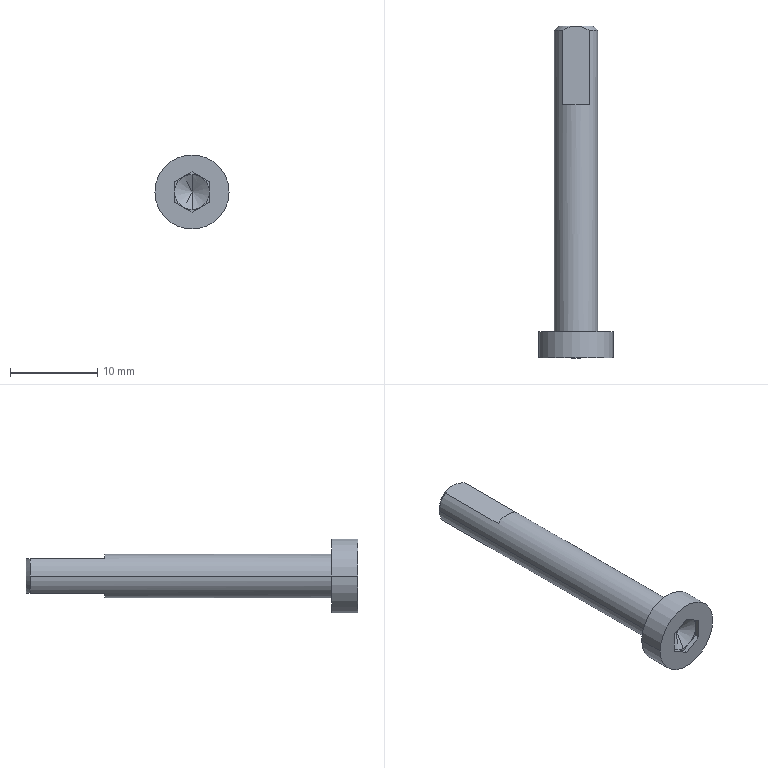Component | SolidWorks | 18M5-L35StainlessSteelScrew-1 | 1 solid | 28 faces | box 8.5 x 38 x 8.5 mm | volume 826 mm3 | plane 19 | cone 5 | cylinder 4 | commonest cylinder face diameters 5 x2 8.5 x2 | material SUS304
STEP:
#1=COLOUR_RGB('',0.7922,0.8196,0.9333);
#2=FILL_AREA_STYLE_COLOUR('',#1);
#3=FILL_AREA_STYLE('',(#2));
#4=SURFACE_STYLE_FILL_AREA(#3);
#5=SURFACE_SIDE_STYLE('',(#4));
#6=SURFACE_STYLE_USAGE(.BOTH.,#5);
#7=PRESENTATION_STYLE_ASSIGNMENT((#6));
#8=CARTESIAN_POINT('',(-0.5354,0.004919,3.11));
#9=VERTEX_POINT('',#8);
#10=CARTESIAN_POINT('',(-0.5354,-0.04054,3.031));
#11=VERTEX_POINT('',#10);
#12=CARTESIAN_POINT('',(-0.5354,-0.04054,3.031));
#13=DIRECTION('',(0.,-0.5,-0.866));
#14=VECTOR('',#13,39.37);
#15=LINE('',#12,#14);
#16=EDGE_CURVE('',#9,#11,#15,.T.);
#17=ORIENTED_EDGE('',*,*,#16,.F.);
#18=CARTESIAN_POINT('',(-0.5354,-0.04054,3.189));
#19=VERTEX_POINT('',#18);
#20=CARTESIAN_POINT('',(-0.5354,-0.04054,3.189));
#21=DIRECTION('',(0.,-0.5,0.866));
#22=VECTOR('',#21,39.37);
#23=LINE('',#20,#22);
#24=EDGE_CURVE('',#9,#19,#23,.T.);
#25=ORIENTED_EDGE('',*,*,#24,.T.);
#26=CARTESIAN_POINT('',(-0.5748,-0.04054,3.178));
#27=VERTEX_POINT('',#26);
#28=CARTESIAN_POINT('',(-0.5354,-0.04054,3.11));
#29=DIRECTION('',(-0.,1.,-0.));
#30=DIRECTION('',(0.,-0.,-1.));
#31=AXIS2_PLACEMENT_3D('',#28,#29,#30);
#32=CIRCLE('',#31,0.07874);
#33=EDGE_CURVE('',#27,#19,#32,.T.);
#34=ORIENTED_EDGE('',*,*,#33,.F.);
#35=CARTESIAN_POINT('',(-0.6142,-0.04054,3.11));
#36=VERTEX_POINT('',#35);
#37=CARTESIAN_POINT('',(-0.5354,-0.04054,3.11));
#38=DIRECTION('',(-0.,1.,-0.));
#39=DIRECTION('',(-0.,-0.,-1.));
#40=AXIS2_PLACEMENT_3D('',#37,#38,#39);
#41=CIRCLE('',#40,0.07874);
#42=EDGE_CURVE('',#36,#27,#41,.T.);
#43=ORIENTED_EDGE('',*,*,#42,.F.);
#44=CARTESIAN_POINT('',(-0.5748,-0.04054,3.042));
#45=VERTEX_POINT('',#44);
#46=CARTESIAN_POINT('',(-0.5354,-0.04054,3.11));
#47=DIRECTION('',(-0.,1.,-0.));
#48=DIRECTION('',(0.,-0.,-1.));
#49=AXIS2_PLACEMENT_3D('',#46,#47,#48);
#50=CIRCLE('',#49,0.07874);
#51=EDGE_CURVE('',#45,#36,#50,.T.);
#52=ORIENTED_EDGE('',*,*,#51,.F.);
#53=CARTESIAN_POINT('',(-0.5354,-0.04054,3.11));
#54=DIRECTION('',(-0.,1.,-0.));
#55=DIRECTION('',(0.,-0.,-1.));
#56=AXIS2_PLACEMENT_3D('',#53,#54,#55);
#57=CIRCLE('',#56,0.07874);
#58=EDGE_CURVE('',#11,#45,#57,.T.);
#59=ORIENTED_EDGE('',*,*,#58,.F.);
#60=EDGE_LOOP('',(#17,#25,#34,#43,#52,#59));
#61=FACE_OUTER_BOUND('',#60,.T.);
#62=CARTESIAN_POINT('',(-0.5354,-0.04054,3.11));
#63=DIRECTION('',(0.,-1.,0.));
#64=DIRECTION('',(0.,-0.,-1.));
#65=AXIS2_PLACEMENT_3D('',#62,#63,#64);
#66=CONICAL_SURFACE('',#65,0.07874,1.047);
#67=ADVANCED_FACE('',(#61),#66,.F.);
#68=CARTESIAN_POINT('',(-0.5945,1.417,3.189));
#69=VERTEX_POINT('',#68);
#70=CARTESIAN_POINT('',(-0.6338,1.417,3.11));
#71=VERTEX_POINT('',#70);
#72=CARTESIAN_POINT('',(-0.5354,1.417,3.11));
#73=DIRECTION('',(0.,-1.,0.));
#74=DIRECTION('',(1.,0.,0.));
#75=AXIS2_PLACEMENT_3D('',#72,#73,#74);
#76=CIRCLE('',#75,0.09843);
#77=EDGE_CURVE('',#69,#71,#76,.T.);
#78=ORIENTED_EDGE('',*,*,#77,.T.);
#79=CARTESIAN_POINT('',(-0.6338,0.05788,3.11));
#80=VERTEX_POINT('',#79);
#81=CARTESIAN_POINT('',(-0.6338,1.436,3.11));
#82=DIRECTION('',(0.,-1.,0.));
#83=VECTOR('',#82,39.37);
#84=LINE('',#81,#83);
#85=EDGE_CURVE('',#71,#80,#84,.T.);
#86=ORIENTED_EDGE('',*,*,#85,.T.);
#87=CARTESIAN_POINT('',(-0.437,0.05788,3.11));
#88=VERTEX_POINT('',#87);
#89=CARTESIAN_POINT('',(-0.5354,0.05788,3.11));
#90=DIRECTION('',(-0.,1.,-0.));
#91=DIRECTION('',(1.,0.,0.));
#92=AXIS2_PLACEMENT_3D('',#89,#90,#91);
#93=CIRCLE('',#92,0.09843);
#94=EDGE_CURVE('',#80,#88,#93,.T.);
#95=ORIENTED_EDGE('',*,*,#94,.T.);
#96=CARTESIAN_POINT('',(-0.437,1.417,3.11));
#97=VERTEX_POINT('',#96);
#98=CARTESIAN_POINT('',(-0.437,1.436,3.11));
#99=DIRECTION('',(0.,-1.,0.));
#100=VECTOR('',#99,39.37);
#101=LINE('',#98,#100);
#102=EDGE_CURVE('',#97,#88,#101,.T.);
#103=ORIENTED_EDGE('',*,*,#102,.F.);
#104=CARTESIAN_POINT('',(-0.4764,1.417,3.189));
#105=VERTEX_POINT('',#104);
#106=CARTESIAN_POINT('',(-0.5354,1.417,3.11));
#107=DIRECTION('',(0.,-1.,0.));
#108=DIRECTION('',(1.,0.,0.));
#109=AXIS2_PLACEMENT_3D('',#106,#107,#108);
#110=CIRCLE('',#109,0.09843);
#111=EDGE_CURVE('',#97,#105,#110,.T.);
#112=ORIENTED_EDGE('',*,*,#111,.T.);
#113=CARTESIAN_POINT('',(-0.4764,1.082,3.189));
#114=VERTEX_POINT('',#113);
#115=CARTESIAN_POINT('',(-0.4764,1.082,3.189));
#116=DIRECTION('',(-0.,1.,-0.));
#117=VECTOR('',#116,39.37);
#118=LINE('',#115,#117);
#119=EDGE_CURVE('',#114,#105,#118,.T.);
#120=ORIENTED_EDGE('',*,*,#119,.F.);
#121=CARTESIAN_POINT('',(-0.5945,1.082,3.189));
#122=VERTEX_POINT('',#121);
#123=CARTESIAN_POINT('',(-0.5354,1.082,3.11));
#124=DIRECTION('',(-0.,1.,-0.));
#125=DIRECTION('',(-1.,0.,0.));
#126=AXIS2_PLACEMENT_3D('',#123,#124,#125);
#127=CIRCLE('',#126,0.09843);
#128=EDGE_CURVE('',#122,#114,#127,.T.);
#129=ORIENTED_EDGE('',*,*,#128,.F.);
#130=CARTESIAN_POINT('',(-0.5945,1.082,3.189));
#131=DIRECTION('',(-0.,1.,-0.));
#132=VECTOR('',#131,39.37);
#133=LINE('',#130,#132);
#134=EDGE_CURVE('',#122,#69,#133,.T.);
#135=ORIENTED_EDGE('',*,*,#134,.T.);
#136=EDGE_LOOP('',(#78,#86,#95,#103,#112,#120,#129,#135));
#137=FACE_OUTER_BOUND('',#136,.T.);
#138=CARTESIAN_POINT('',(-0.5354,1.436,3.11));
#139=DIRECTION('',(0.,-1.,0.));
#140=DIRECTION('',(1.,0.,0.));
#141=AXIS2_PLACEMENT_3D('',#138,#139,#140);
#142=CYLINDRICAL_SURFACE('',#141,0.09843);
#143=ADVANCED_FACE('',(#137),#142,.T.);
#144=CARTESIAN_POINT('',(-0.5277,1.436,3.031));
#145=VERTEX_POINT('',#144);
#146=CARTESIAN_POINT('',(-0.4563,1.436,3.11));
#147=VERTEX_POINT('',#146);
#148=CARTESIAN_POINT('',(-0.5354,1.436,3.11));
#149=DIRECTION('',(0.,-1.,0.));
#150=DIRECTION('',(1.,0.,0.));
#151=AXIS2_PLACEMENT_3D('',#148,#149,#150);
#152=CIRCLE('',#151,0.07911);
#153=EDGE_CURVE('',#145,#147,#152,.T.);
#154=ORIENTED_EDGE('',*,*,#153,.T.);
#155=CARTESIAN_POINT('',(-0.437,1.417,3.11));
#156=DIRECTION('',(0.7071,-0.7071,0.));
#157=VECTOR('',#156,39.37);
#158=LINE('',#155,#157);
#159=EDGE_CURVE('',#147,#97,#158,.T.);
#160=ORIENTED_EDGE('',*,*,#159,.T.);
#161=CARTESIAN_POINT('',(-0.4764,1.417,3.031));
#162=VERTEX_POINT('',#161);
#163=CARTESIAN_POINT('',(-0.5354,1.417,3.11));
#164=DIRECTION('',(0.,-1.,0.));
#165=DIRECTION('',(1.,0.,0.));
#166=AXIS2_PLACEMENT_3D('',#163,#164,#165);
#167=CIRCLE('',#166,0.09843);
#168=EDGE_CURVE('',#162,#97,#167,.T.);
#169=ORIENTED_EDGE('',*,*,#168,.F.);
#170=CARTESIAN_POINT('',(-0.5277,1.436,3.031));
#171=CARTESIAN_POINT('',(-0.5185,1.435,3.031));
#172=CARTESIAN_POINT('',(-0.5096,1.432,3.031));
#173=CARTESIAN_POINT('',(-0.4924,1.426,3.031));
#174=CARTESIAN_POINT('',(-0.4842,1.421,3.031));
#175=CARTESIAN_POINT('',(-0.4764,1.417,3.031));
#176=B_SPLINE_CURVE_WITH_KNOTS('',3,(#170,#171,#172,#173,#174,#175),.UNSPECIFIED.,.F.,.F.,(4,2,4),(0.004086,0.004787,0.005487),.UNSPECIFIED.);
#177=EDGE_CURVE('',#145,#162,#176,.T.);
#178=ORIENTED_EDGE('',*,*,#177,.F.);
#179=EDGE_LOOP('',(#154,#160,#169,#178));
#180=FACE_OUTER_BOUND('',#179,.T.);
#181=CARTESIAN_POINT('',(-0.5354,1.417,3.11));
#182=DIRECTION('',(0.,-1.,0.));
#183=DIRECTION('',(1.,0.,0.));
#184=AXIS2_PLACEMENT_3D('',#181,#182,#183);
#185=CONICAL_SURFACE('',#184,0.09843,0.7854);
#186=ADVANCED_FACE('',(#180),#185,.T.);
#187=CARTESIAN_POINT('',(-0.3681,0.05788,3.11));
#188=VERTEX_POINT('',#187);
#189=CARTESIAN_POINT('',(-0.7027,0.05788,3.11));
#190=VERTEX_POINT('',#189);
#191=CARTESIAN_POINT('',(-0.5354,0.05788,3.11));
#192=DIRECTION('',(0.,-1.,0.));
#193=DIRECTION('',(1.,0.,0.));
#194=AXIS2_PLACEMENT_3D('',#191,#192,#193);
#195=CIRCLE('',#194,0.1673);
#196=EDGE_CURVE('',#188,#190,#195,.T.);
#197=ORIENTED_EDGE('',*,*,#196,.T.);
#198=CARTESIAN_POINT('',(-0.7027,-0.06023,3.11));
#199=VERTEX_POINT('',#198);
#200=CARTESIAN_POINT('',(-0.7027,0.05788,3.11));
#201=DIRECTION('',(0.,-1.,0.));
#202=VECTOR('',#201,39.37);
#203=LINE('',#200,#202);
#204=EDGE_CURVE('',#190,#199,#203,.T.);
#205=ORIENTED_EDGE('',*,*,#204,.T.);
#206=CARTESIAN_POINT('',(-0.3681,-0.06023,3.11));
#207=VERTEX_POINT('',#206);
#208=CARTESIAN_POINT('',(-0.5354,-0.06023,3.11));
#209=DIRECTION('',(0.,-1.,0.));
#210=DIRECTION('',(1.,0.,0.));
#211=AXIS2_PLACEMENT_3D('',#208,#209,#210);
#212=CIRCLE('',#211,0.1673);
#213=EDGE_CURVE('',#207,#199,#212,.T.);
#214=ORIENTED_EDGE('',*,*,#213,.F.);
#215=CARTESIAN_POINT('',(-0.3681,0.05788,3.11));
#216=DIRECTION('',(0.,-1.,0.));
#217=VECTOR('',#216,39.37);
#218=LINE('',#215,#217);
#219=EDGE_CURVE('',#188,#207,#218,.T.);
#220=ORIENTED_EDGE('',*,*,#219,.F.);
#221=EDGE_LOOP('',(#197,#205,#214,#220));
#222=FACE_OUTER_BOUND('',#221,.T.);
#223=CARTESIAN_POINT('',(-0.5354,0.05788,3.11));
#224=DIRECTION('',(0.,-1.,0.));
#225=DIRECTION('',(1.,0.,0.));
#226=AXIS2_PLACEMENT_3D('',#223,#224,#225);
#227=CYLINDRICAL_SURFACE('',#226,0.1673);
#228=ADVANCED_FACE('',(#222),#227,.T.);
#229=ORIENTED_EDGE('',*,*,#204,.F.);
#230=CARTESIAN_POINT('',(-0.5354,0.05788,3.11));
#231=DIRECTION('',(0.,-1.,0.));
#232=DIRECTION('',(1.,0.,0.));
#233=AXIS2_PLACEMENT_3D('',#230,#231,#232);
#234=CIRCLE('',#233,0.1673);
#235=EDGE_CURVE('',#190,#188,#234,.T.);
#236=ORIENTED_EDGE('',*,*,#235,.T.);
#237=ORIENTED_EDGE('',*,*,#219,.T.);
#238=CARTESIAN_POINT('',(-0.5354,-0.06023,3.11));
#239=DIRECTION('',(0.,-1.,0.));
#240=DIRECTION('',(1.,0.,0.));
#241=AXIS2_PLACEMENT_3D('',#238,#239,#240);
#242=CIRCLE('',#241,0.1673);
#243=EDGE_CURVE('',#199,#207,#242,.T.);
#244=ORIENTED_EDGE('',*,*,#243,.F.);
#245=EDGE_LOOP('',(#229,#236,#237,#244));
#246=FACE_OUTER_BOUND('',#245,.T.);
#247=CARTESIAN_POINT('',(-0.5354,0.05788,3.11));
#248=DIRECTION('',(0.,-1.,0.));
#249=DIRECTION('',(1.,0.,0.));
#250=AXIS2_PLACEMENT_3D('',#247,#248,#249);
#251=CYLINDRICAL_SURFACE('',#250,0.1673);
#252=ADVANCED_FACE('',(#246),#251,.T.);
#253=CARTESIAN_POINT('',(-0.5945,1.417,3.031));
#254=VERTEX_POINT('',#253);
#255=CARTESIAN_POINT('',(-0.5431,1.436,3.031));
#256=VERTEX_POINT('',#255);
#257=CARTESIAN_POINT('',(-0.5945,1.417,3.031));
#258=CARTESIAN_POINT('',(-0.5866,1.421,3.031));
#259=CARTESIAN_POINT('',(-0.5785,1.426,3.031));
#260=CARTESIAN_POINT('',(-0.5613,1.432,3.031));
#261=CARTESIAN_POINT('',(-0.5523,1.435,3.031));
#262=CARTESIAN_POINT('',(-0.5431,1.436,3.031));
#263=B_SPLINE_CURVE_WITH_KNOTS('',3,(#257,#258,#259,#260,#261,#262),.UNSPECIFIED.,.F.,.F.,(4,2,4),(0.002291,0.002994,0.003697),.UNSPECIFIED.);
#264=EDGE_CURVE('',#254,#256,#263,.T.);
#265=ORIENTED_EDGE('',*,*,#264,.F.);
#266=CARTESIAN_POINT('',(-0.5354,1.417,3.11));
#267=DIRECTION('',(0.,-1.,0.));
#268=DIRECTION('',(1.,0.,0.));
#269=AXIS2_PLACEMENT_3D('',#266,#267,#268);
#270=CIRCLE('',#269,0.09843);
#271=EDGE_CURVE('',#71,#254,#270,.T.);
#272=ORIENTED_EDGE('',*,*,#271,.F.);
#273=ORIENTED_EDGE('',*,*,#77,.F.);
#274=CARTESIAN_POINT('',(-0.5431,1.436,3.189));
#275=VERTEX_POINT('',#274);
#276=CARTESIAN_POINT('',(-0.5431,1.436,3.189));
#277=CARTESIAN_POINT('',(-0.5524,1.435,3.189));
#278=CARTESIAN_POINT('',(-0.5612,1.432,3.189));
#279=CARTESIAN_POINT('',(-0.5785,1.426,3.189));
#280=CARTESIAN_POINT('',(-0.5866,1.421,3.189));
#281=CARTESIAN_POINT('',(-0.5945,1.417,3.189));
#282=B_SPLINE_CURVE_WITH_KNOTS('',3,(#276,#277,#278,#279,#280,#281),.UNSPECIFIED.,.F.,.F.,(4,2,4),(0.004086,0.004787,0.005487),.UNSPECIFIED.);
#283=EDGE_CURVE('',#275,#69,#282,.T.);
#284=ORIENTED_EDGE('',*,*,#283,.F.);
#285=CARTESIAN_POINT('',(-0.5354,1.436,3.11));
#286=DIRECTION('',(0.,-1.,0.));
#287=DIRECTION('',(1.,0.,0.));
#288=AXIS2_PLACEMENT_3D('',#285,#286,#287);
#289=CIRCLE('',#288,0.07911);
#290=EDGE_CURVE('',#275,#256,#289,.T.);
#291=ORIENTED_EDGE('',*,*,#290,.T.);
#292=EDGE_LOOP('',(#265,#272,#273,#284,#291));
#293=FACE_OUTER_BOUND('',#292,.T.);
#294=CARTESIAN_POINT('',(-0.5354,1.417,3.11));
#295=DIRECTION('',(0.,-1.,0.));
#296=DIRECTION('',(1.,0.,0.));
#297=AXIS2_PLACEMENT_3D('',#294,#295,#296);
#298=CONICAL_SURFACE('',#297,0.09843,0.7854);
#299=ADVANCED_FACE('',(#293),#298,.T.);
#300=ORIENTED_EDGE('',*,*,#85,.F.);
#301=ORIENTED_EDGE('',*,*,#271,.T.);
#302=CARTESIAN_POINT('',(-0.5945,1.082,3.031));
#303=VERTEX_POINT('',#302);
#304=CARTESIAN_POINT('',(-0.5945,1.082,3.031));
#305=DIRECTION('',(-0.,1.,-0.));
#306=VECTOR('',#305,39.37);
#307=LINE('',#304,#306);
#308=EDGE_CURVE('',#303,#254,#307,.T.);
#309=ORIENTED_EDGE('',*,*,#308,.F.);
#310=CARTESIAN_POINT('',(-0.4764,1.082,3.031));
#311=VERTEX_POINT('',#310);
#312=CARTESIAN_POINT('',(-0.5354,1.082,3.11));
#313=DIRECTION('',(-0.,1.,-0.));
#314=DIRECTION('',(-1.,0.,0.));
#315=AXIS2_PLACEMENT_3D('',#312,#313,#314);
#316=CIRCLE('',#315,0.09843);
#317=EDGE_CURVE('',#311,#303,#316,.T.);
#318=ORIENTED_EDGE('',*,*,#317,.F.);
#319=CARTESIAN_POINT('',(-0.4764,1.082,3.031));
#320=DIRECTION('',(-0.,1.,-0.));
#321=VECTOR('',#320,39.37);
#322=LINE('',#319,#321);
#323=EDGE_CURVE('',#311,#162,#322,.T.);
#324=ORIENTED_EDGE('',*,*,#323,.T.);
#325=ORIENTED_EDGE('',*,*,#168,.T.);
#326=ORIENTED_EDGE('',*,*,#102,.T.);
#327=CARTESIAN_POINT('',(-0.5354,0.05788,3.11));
#328=DIRECTION('',(-0.,1.,-0.));
#329=DIRECTION('',(1.,0.,0.));
#330=AXIS2_PLACEMENT_3D('',#327,#328,#329);
#331=CIRCLE('',#330,0.09843);
#332=EDGE_CURVE('',#88,#80,#331,.T.);
#333=ORIENTED_EDGE('',*,*,#332,.T.);
#334=EDGE_LOOP('',(#300,#301,#309,#318,#324,#325,#326,#333));
#335=FACE_OUTER_BOUND('',#334,.T.);
#336=CARTESIAN_POINT('',(-0.5354,1.436,3.11));
#337=DIRECTION('',(0.,-1.,0.));
#338=DIRECTION('',(1.,0.,0.));
#339=AXIS2_PLACEMENT_3D('',#336,#337,#338);
#340=CYLINDRICAL_SURFACE('',#339,0.09843);
#341=ADVANCED_FACE('',(#335),#340,.T.);
#342=ORIENTED_EDGE('',*,*,#196,.F.);
#343=ORIENTED_EDGE('',*,*,#235,.F.);
#344=EDGE_LOOP('',(#342,#343));
#345=FACE_OUTER_BOUND('',#344,.T.);
#346=ORIENTED_EDGE('',*,*,#332,.F.);
#347=ORIENTED_EDGE('',*,*,#94,.F.);
#348=EDGE_LOOP('',(#346,#347));
#349=FACE_BOUND('',#348,.T.);
#350=CARTESIAN_POINT('',(-0.5354,0.05788,3.278));
#351=DIRECTION('',(0.,-1.,0.));
#352=DIRECTION('',(1.,0.,0.));
#353=AXIS2_PLACEMENT_3D('',#350,#351,#352);
#354=PLANE('',#353);
#355=ADVANCED_FACE('',(#345,#349),#354,.F.);
#356=ORIENTED_EDGE('',*,*,#159,.F.);
#357=CARTESIAN_POINT('',(-0.5277,1.436,3.189));
#358=VERTEX_POINT('',#357);
#359=CARTESIAN_POINT('',(-0.5354,1.436,3.11));
#360=DIRECTION('',(0.,-1.,0.));
#361=DIRECTION('',(1.,0.,0.));
#362=AXIS2_PLACEMENT_3D('',#359,#360,#361);
#363=CIRCLE('',#362,0.07911);
#364=EDGE_CURVE('',#147,#358,#363,.T.);
#365=ORIENTED_EDGE('',*,*,#364,.T.);
#366=CARTESIAN_POINT('',(-0.4764,1.417,3.189));
#367=CARTESIAN_POINT('',(-0.4842,1.421,3.189));
#368=CARTESIAN_POINT('',(-0.4923,1.426,3.189));
#369=CARTESIAN_POINT('',(-0.5095,1.432,3.189));
#370=CARTESIAN_POINT('',(-0.5186,1.435,3.189));
#371=CARTESIAN_POINT('',(-0.5277,1.436,3.189));
#372=B_SPLINE_CURVE_WITH_KNOTS('',3,(#366,#367,#368,#369,#370,#371),.UNSPECIFIED.,.F.,.F.,(4,2,4),(0.002291,0.002994,0.003697),.UNSPECIFIED.);
#373=EDGE_CURVE('',#105,#358,#372,.T.);
#374=ORIENTED_EDGE('',*,*,#373,.F.);
#375=ORIENTED_EDGE('',*,*,#111,.F.);
#376=EDGE_LOOP('',(#356,#365,#374,#375));
#377=FACE_OUTER_BOUND('',#376,.T.);
#378=CARTESIAN_POINT('',(-0.5354,1.417,3.11));
#379=DIRECTION('',(0.,-1.,0.));
#380=DIRECTION('',(1.,0.,0.));
#381=AXIS2_PLACEMENT_3D('',#378,#379,#380);
#382=CONICAL_SURFACE('',#381,0.09843,0.7854);
#383=ADVANCED_FACE('',(#377),#382,.T.);
#384=ORIENTED_EDGE('',*,*,#153,.F.);
#385=CARTESIAN_POINT('',(-0.4764,1.436,3.031));
#386=DIRECTION('',(1.,0.,0.));
#387=VECTOR('',#386,39.37);
#388=LINE('',#385,#387);
#389=EDGE_CURVE('',#256,#145,#388,.T.);
#390=ORIENTED_EDGE('',*,*,#389,.F.);
#391=ORIENTED_EDGE('',*,*,#290,.F.);
#392=CARTESIAN_POINT('',(-0.4764,1.436,3.189));
#393=DIRECTION('',(-1.,-0.,0.));
#394=VECTOR('',#393,39.37);
#395=LINE('',#392,#394);
#396=EDGE_CURVE('',#358,#275,#395,.T.);
#397=ORIENTED_EDGE('',*,*,#396,.F.);
#398=ORIENTED_EDGE('',*,*,#364,.F.);
#399=EDGE_LOOP('',(#384,#390,#391,#397,#398));
#400=FACE_OUTER_BOUND('',#399,.T.);
#401=CARTESIAN_POINT('',(-0.5354,1.436,3.189));
#402=DIRECTION('',(0.,-1.,0.));
#403=DIRECTION('',(1.,0.,0.));
#404=AXIS2_PLACEMENT_3D('',#401,#402,#403);
#405=PLANE('',#404);
#406=ADVANCED_FACE('',(#400),#405,.F.);
#407=ORIENTED_EDGE('',*,*,#373,.T.);
#408=ORIENTED_EDGE('',*,*,#396,.T.);
#409=ORIENTED_EDGE('',*,*,#283,.T.);
#410=ORIENTED_EDGE('',*,*,#134,.F.);
#411=CARTESIAN_POINT('',(-0.4764,1.082,3.189));
#412=DIRECTION('',(-1.,-0.,0.));
#413=VECTOR('',#412,39.37);
#414=LINE('',#411,#413);
#415=EDGE_CURVE('',#114,#122,#414,.T.);
#416=ORIENTED_EDGE('',*,*,#415,.F.);
#417=ORIENTED_EDGE('',*,*,#119,.T.);
#418=EDGE_LOOP('',(#407,#408,#409,#410,#416,#417));
#419=FACE_OUTER_BOUND('',#418,.T.);
#420=CARTESIAN_POINT('',(-0.4764,1.082,3.189));
#421=DIRECTION('',(-0.,-0.,-1.));
#422=DIRECTION('',(-0.,1.,-0.));
#423=AXIS2_PLACEMENT_3D('',#420,#421,#422);
#424=PLANE('',#423);
#425=ADVANCED_FACE('',(#419),#424,.F.);
#426=ORIENTED_EDGE('',*,*,#128,.T.);
#427=ORIENTED_EDGE('',*,*,#415,.T.);
#428=EDGE_LOOP('',(#426,#427));
#429=FACE_OUTER_BOUND('',#428,.T.);
#430=CARTESIAN_POINT('',(-0.5354,1.082,3.11));
#431=DIRECTION('',(-0.,1.,-0.));
#432=DIRECTION('',(-1.,-0.,0.));
#433=AXIS2_PLACEMENT_3D('',#430,#431,#432);
#434=PLANE('',#433);
#435=ADVANCED_FACE('',(#429),#434,.T.);
#436=ORIENTED_EDGE('',*,*,#264,.T.);
#437=ORIENTED_EDGE('',*,*,#389,.T.);
#438=ORIENTED_EDGE('',*,*,#177,.T.);
#439=ORIENTED_EDGE('',*,*,#323,.F.);
#440=CARTESIAN_POINT('',(-0.4764,1.082,3.031));
#441=DIRECTION('',(1.,0.,0.));
#442=VECTOR('',#441,39.37);
#443=LINE('',#440,#442);
#444=EDGE_CURVE('',#303,#311,#443,.T.);
#445=ORIENTED_EDGE('',*,*,#444,.F.);
#446=ORIENTED_EDGE('',*,*,#308,.T.);
#447=EDGE_LOOP('',(#436,#437,#438,#439,#445,#446));
#448=FACE_OUTER_BOUND('',#447,.T.);
#449=CARTESIAN_POINT('',(-0.4764,1.082,3.031));
#450=DIRECTION('',(0.,0.,1.));
#451=DIRECTION('',(0.,-1.,0.));
#452=AXIS2_PLACEMENT_3D('',#449,#450,#451);
#453=PLANE('',#452);
#454=ADVANCED_FACE('',(#448),#453,.F.);
#455=ORIENTED_EDGE('',*,*,#317,.T.);
#456=ORIENTED_EDGE('',*,*,#444,.T.);
#457=EDGE_LOOP('',(#455,#456));
#458=FACE_OUTER_BOUND('',#457,.T.);
#459=CARTESIAN_POINT('',(-0.5354,1.082,3.11));
#460=DIRECTION('',(-0.,1.,-0.));
#461=DIRECTION('',(-1.,-0.,0.));
#462=AXIS2_PLACEMENT_3D('',#459,#460,#461);
#463=PLANE('',#462);
#464=ADVANCED_FACE('',(#458),#463,.T.);
#465=ORIENTED_EDGE('',*,*,#213,.T.);
#466=ORIENTED_EDGE('',*,*,#243,.T.);
#467=EDGE_LOOP('',(#465,#466));
#468=FACE_OUTER_BOUND('',#467,.T.);
#469=CARTESIAN_POINT('',(-0.4567,-0.06023,3.156));
#470=VERTEX_POINT('',#469);
#471=CARTESIAN_POINT('',(-0.4567,-0.06023,3.065));
#472=VERTEX_POINT('',#471);
#473=CARTESIAN_POINT('',(-0.4567,-0.06023,3.065));
#474=DIRECTION('',(0.,-0.,-1.));
#475=VECTOR('',#474,39.37);
#476=LINE('',#473,#475);
#477=EDGE_CURVE('',#470,#472,#476,.T.);
#478=ORIENTED_EDGE('',*,*,#477,.T.);
#479=CARTESIAN_POINT('',(-0.5354,-0.06023,3.019));
#480=VERTEX_POINT('',#479);
#481=CARTESIAN_POINT('',(-0.5354,-0.06023,3.019));
#482=DIRECTION('',(-0.866,-0.,-0.5));
#483=VECTOR('',#482,39.37);
#484=LINE('',#481,#483);
#485=EDGE_CURVE('',#472,#480,#484,.T.);
#486=ORIENTED_EDGE('',*,*,#485,.T.);
#487=CARTESIAN_POINT('',(-0.6142,-0.06023,3.065));
#488=VERTEX_POINT('',#487);
#489=CARTESIAN_POINT('',(-0.6142,-0.06023,3.065));
#490=DIRECTION('',(-0.866,-0.,0.5));
#491=VECTOR('',#490,39.37);
#492=LINE('',#489,#491);
#493=EDGE_CURVE('',#480,#488,#492,.T.);
#494=ORIENTED_EDGE('',*,*,#493,.T.);
#495=CARTESIAN_POINT('',(-0.6142,-0.06023,3.156));
#496=VERTEX_POINT('',#495);
#497=CARTESIAN_POINT('',(-0.6142,-0.06023,3.156));
#498=DIRECTION('',(0.,0.,1.));
#499=VECTOR('',#498,39.37);
#500=LINE('',#497,#499);
#501=EDGE_CURVE('',#488,#496,#500,.T.);
#502=ORIENTED_EDGE('',*,*,#501,.T.);
#503=CARTESIAN_POINT('',(-0.5354,-0.06023,3.201));
#504=VERTEX_POINT('',#503);
#505=CARTESIAN_POINT('',(-0.5354,-0.06023,3.201));
#506=DIRECTION('',(0.866,0.,0.5));
#507=VECTOR('',#506,39.37);
#508=LINE('',#505,#507);
#509=EDGE_CURVE('',#496,#504,#508,.T.);
#510=ORIENTED_EDGE('',*,*,#509,.T.);
#511=CARTESIAN_POINT('',(-0.4567,-0.06023,3.156));
#512=DIRECTION('',(0.866,0.,-0.5));
#513=VECTOR('',#512,39.37);
#514=LINE('',#511,#513);
#515=EDGE_CURVE('',#504,#470,#514,.T.);
#516=ORIENTED_EDGE('',*,*,#515,.T.);
#517=EDGE_LOOP('',(#478,#486,#494,#502,#510,#516));
#518=FACE_BOUND('',#517,.T.);
#519=CARTESIAN_POINT('',(-0.5354,-0.06023,3.11));
#520=DIRECTION('',(0.,-1.,0.));
#521=DIRECTION('',(1.,0.,0.));
#522=AXIS2_PLACEMENT_3D('',#519,#520,#521);
#523=PLANE('',#522);
#524=ADVANCED_FACE('',(#468,#518),#523,.T.);
#525=ORIENTED_EDGE('',*,*,#24,.F.);
#526=ORIENTED_EDGE('',*,*,#16,.T.);
#527=CARTESIAN_POINT('',(-0.496,-0.04054,3.042));
#528=VERTEX_POINT('',#527);
#529=CARTESIAN_POINT('',(-0.5354,-0.04054,3.11));
#530=DIRECTION('',(-0.,1.,-0.));
#531=DIRECTION('',(0.,-0.,-1.));
#532=AXIS2_PLACEMENT_3D('',#529,#530,#531);
#533=CIRCLE('',#532,0.07874);
#534=EDGE_CURVE('',#528,#11,#533,.T.);
#535=ORIENTED_EDGE('',*,*,#534,.F.);
#536=CARTESIAN_POINT('',(-0.4567,-0.04054,3.11));
#537=VERTEX_POINT('',#536);
#538=CARTESIAN_POINT('',(-0.5354,-0.04054,3.11));
#539=DIRECTION('',(-0.,1.,-0.));
#540=DIRECTION('',(-0.,-0.,-1.));
#541=AXIS2_PLACEMENT_3D('',#538,#539,#540);
#542=CIRCLE('',#541,0.07874);
#543=EDGE_CURVE('',#537,#528,#542,.T.);
#544=ORIENTED_EDGE('',*,*,#543,.F.);
#545=CARTESIAN_POINT('',(-0.496,-0.04054,3.178));
#546=VERTEX_POINT('',#545);
#547=CARTESIAN_POINT('',(-0.5354,-0.04054,3.11));
#548=DIRECTION('',(-0.,1.,-0.));
#549=DIRECTION('',(0.,-0.,-1.));
#550=AXIS2_PLACEMENT_3D('',#547,#548,#549);
#551=CIRCLE('',#550,0.07874);
#552=EDGE_CURVE('',#546,#537,#551,.T.);
#553=ORIENTED_EDGE('',*,*,#552,.F.);
#554=CARTESIAN_POINT('',(-0.5354,-0.04054,3.11));
#555=DIRECTION('',(-0.,1.,-0.));
#556=DIRECTION('',(-0.,-0.,-1.));
#557=AXIS2_PLACEMENT_3D('',#554,#555,#556);
#558=CIRCLE('',#557,0.07874);
#559=EDGE_CURVE('',#19,#546,#558,.T.);
#560=ORIENTED_EDGE('',*,*,#559,.F.);
#561=EDGE_LOOP('',(#525,#526,#535,#544,#553,#560));
#562=FACE_OUTER_BOUND('',#561,.T.);
#563=CARTESIAN_POINT('',(-0.5354,-0.04054,3.11));
#564=DIRECTION('',(0.,-1.,0.));
#565=DIRECTION('',(0.,-0.,-1.));
#566=AXIS2_PLACEMENT_3D('',#563,#564,#565);
#567=CONICAL_SURFACE('',#566,0.07874,1.047);
#568=ADVANCED_FACE('',(#562),#567,.F.);
#569=ORIENTED_EDGE('',*,*,#552,.T.);
#570=CARTESIAN_POINT('',(-0.4567,-0.04054,3.156));
#571=VERTEX_POINT('',#570);
#572=CARTESIAN_POINT('',(-0.4567,-0.04054,3.065));
#573=DIRECTION('',(0.,0.,1.));
#574=VECTOR('',#573,39.37);
#575=LINE('',#572,#574);
#576=EDGE_CURVE('',#537,#571,#575,.T.);
#577=ORIENTED_EDGE('',*,*,#576,.T.);
#578=CARTESIAN_POINT('',(-0.4567,-0.04054,3.156));
#579=DIRECTION('',(-0.866,-0.,0.5));
#580=VECTOR('',#579,39.37);
#581=LINE('',#578,#580);
#582=EDGE_CURVE('',#571,#546,#581,.T.);
#583=ORIENTED_EDGE('',*,*,#582,.T.);
#584=EDGE_LOOP('',(#569,#577,#583));
#585=FACE_OUTER_BOUND('',#584,.T.);
#586=CARTESIAN_POINT('',(-0.5354,-0.04054,3.11));
#587=DIRECTION('',(0.,-1.,0.));
#588=DIRECTION('',(1.,0.,0.));
#589=AXIS2_PLACEMENT_3D('',#586,#587,#588);
#590=PLANE('',#589);
#591=ADVANCED_FACE('',(#585),#590,.T.);
#592=ORIENTED_EDGE('',*,*,#33,.T.);
#593=ORIENTED_EDGE('',*,*,#559,.T.);
#594=CARTESIAN_POINT('',(-0.5354,-0.04054,3.201));
#595=VERTEX_POINT('',#594);
#596=CARTESIAN_POINT('',(-0.496,-0.04054,3.178));
#597=DIRECTION('',(-0.866,-0.,0.5));
#598=VECTOR('',#597,39.37);
#599=LINE('',#596,#598);
#600=EDGE_CURVE('',#546,#595,#599,.T.);
#601=ORIENTED_EDGE('',*,*,#600,.T.);
#602=CARTESIAN_POINT('',(-0.5354,-0.04054,3.201));
#603=DIRECTION('',(-0.866,-0.,-0.5));
#604=VECTOR('',#603,39.37);
#605=LINE('',#602,#604);
#606=EDGE_CURVE('',#595,#27,#605,.T.);
#607=ORIENTED_EDGE('',*,*,#606,.T.);
#608=EDGE_LOOP('',(#592,#593,#601,#607));
#609=FACE_OUTER_BOUND('',#608,.T.);
#610=CARTESIAN_POINT('',(-0.5354,-0.04054,3.11));
#611=DIRECTION('',(0.,-1.,0.));
#612=DIRECTION('',(1.,0.,0.));
#613=AXIS2_PLACEMENT_3D('',#610,#611,#612);
#614=PLANE('',#613);
#615=ADVANCED_FACE('',(#609),#614,.T.);
#616=ORIENTED_EDGE('',*,*,#42,.T.);
#617=CARTESIAN_POINT('',(-0.6142,-0.04054,3.156));
#618=VERTEX_POINT('',#617);
#619=CARTESIAN_POINT('',(-0.5748,-0.04054,3.178));
#620=DIRECTION('',(-0.866,-0.,-0.5));
#621=VECTOR('',#620,39.37);
#622=LINE('',#619,#621);
#623=EDGE_CURVE('',#27,#618,#622,.T.);
#624=ORIENTED_EDGE('',*,*,#623,.T.);
#625=CARTESIAN_POINT('',(-0.6142,-0.04054,3.11));
#626=DIRECTION('',(0.,-0.,-1.));
#627=VECTOR('',#626,39.37);
#628=LINE('',#625,#627);
#629=EDGE_CURVE('',#618,#36,#628,.T.);
#630=ORIENTED_EDGE('',*,*,#629,.T.);
#631=EDGE_LOOP('',(#616,#624,#630));
#632=FACE_OUTER_BOUND('',#631,.T.);
#633=CARTESIAN_POINT('',(-0.5354,-0.04054,3.11));
#634=DIRECTION('',(0.,-1.,0.));
#635=DIRECTION('',(1.,0.,0.));
#636=AXIS2_PLACEMENT_3D('',#633,#634,#635);
#637=PLANE('',#636);
#638=ADVANCED_FACE('',(#632),#637,.T.);
#639=ORIENTED_EDGE('',*,*,#51,.T.);
#640=CARTESIAN_POINT('',(-0.6142,-0.04054,3.065));
#641=VERTEX_POINT('',#640);
#642=CARTESIAN_POINT('',(-0.6142,-0.04054,3.11));
#643=DIRECTION('',(0.,-0.,-1.));
#644=VECTOR('',#643,39.37);
#645=LINE('',#642,#644);
#646=EDGE_CURVE('',#36,#641,#645,.T.);
#647=ORIENTED_EDGE('',*,*,#646,.T.);
#648=CARTESIAN_POINT('',(-0.6142,-0.04054,3.065));
#649=DIRECTION('',(0.866,0.,-0.5));
#650=VECTOR('',#649,39.37);
#651=LINE('',#648,#650);
#652=EDGE_CURVE('',#641,#45,#651,.T.);
#653=ORIENTED_EDGE('',*,*,#652,.T.);
#654=EDGE_LOOP('',(#639,#647,#653));
#655=FACE_OUTER_BOUND('',#654,.T.);
#656=CARTESIAN_POINT('',(-0.5354,-0.04054,3.11));
#657=DIRECTION('',(0.,-1.,0.));
#658=DIRECTION('',(1.,0.,0.));
#659=AXIS2_PLACEMENT_3D('',#656,#657,#658);
#660=PLANE('',#659);
#661=ADVANCED_FACE('',(#655),#660,.T.);
#662=ORIENTED_EDGE('',*,*,#534,.T.);
#663=ORIENTED_EDGE('',*,*,#58,.T.);
#664=CARTESIAN_POINT('',(-0.5354,-0.04054,3.019));
#665=VERTEX_POINT('',#664);
#666=CARTESIAN_POINT('',(-0.5748,-0.04054,3.042));
#667=DIRECTION('',(0.866,0.,-0.5));
#668=VECTOR('',#667,39.37);
#669=LINE('',#666,#668);
#670=EDGE_CURVE('',#45,#665,#669,.T.);
#671=ORIENTED_EDGE('',*,*,#670,.T.);
#672=CARTESIAN_POINT('',(-0.5354,-0.04054,3.019));
#673=DIRECTION('',(0.866,0.,0.5));
#674=VECTOR('',#673,39.37);
#675=LINE('',#672,#674);
#676=EDGE_CURVE('',#665,#528,#675,.T.);
#677=ORIENTED_EDGE('',*,*,#676,.T.);
#678=EDGE_LOOP('',(#662,#663,#671,#677));
#679=FACE_OUTER_BOUND('',#678,.T.);
#680=CARTESIAN_POINT('',(-0.5354,-0.04054,3.11));
#681=DIRECTION('',(0.,-1.,0.));
#682=DIRECTION('',(1.,0.,0.));
#683=AXIS2_PLACEMENT_3D('',#680,#681,#682);
#684=PLANE('',#683);
#685=ADVANCED_FACE('',(#679),#684,.T.);
#686=ORIENTED_EDGE('',*,*,#543,.T.);
#687=CARTESIAN_POINT('',(-0.4567,-0.04054,3.065));
#688=VERTEX_POINT('',#687);
#689=CARTESIAN_POINT('',(-0.496,-0.04054,3.042));
#690=DIRECTION('',(0.866,0.,0.5));
#691=VECTOR('',#690,39.37);
#692=LINE('',#689,#691);
#693=EDGE_CURVE('',#528,#688,#692,.T.);
#694=ORIENTED_EDGE('',*,*,#693,.T.);
#695=CARTESIAN_POINT('',(-0.4567,-0.04054,3.11));
#696=DIRECTION('',(0.,0.,1.));
#697=VECTOR('',#696,39.37);
#698=LINE('',#695,#697);
#699=EDGE_CURVE('',#688,#537,#698,.T.);
#700=ORIENTED_EDGE('',*,*,#699,.T.);
#701=EDGE_LOOP('',(#686,#694,#700));
#702=FACE_OUTER_BOUND('',#701,.T.);
#703=CARTESIAN_POINT('',(-0.5354,-0.04054,3.11));
#704=DIRECTION('',(0.,-1.,0.));
#705=DIRECTION('',(1.,0.,0.));
#706=AXIS2_PLACEMENT_3D('',#703,#704,#705);
#707=PLANE('',#706);
#708=ADVANCED_FACE('',(#702),#707,.T.);
#709=ORIENTED_EDGE('',*,*,#485,.F.);
#710=CARTESIAN_POINT('',(-0.4567,-0.04054,3.065));
#711=DIRECTION('',(0.,-1.,0.));
#712=VECTOR('',#711,39.37);
#713=LINE('',#710,#712);
#714=EDGE_CURVE('',#688,#472,#713,.T.);
#715=ORIENTED_EDGE('',*,*,#714,.F.);
#716=ORIENTED_EDGE('',*,*,#693,.F.);
#717=ORIENTED_EDGE('',*,*,#676,.F.);
#718=CARTESIAN_POINT('',(-0.5354,-0.04054,3.019));
#719=DIRECTION('',(-0.,1.,-0.));
#720=VECTOR('',#719,39.37);
#721=LINE('',#718,#720);
#722=EDGE_CURVE('',#480,#665,#721,.T.);
#723=ORIENTED_EDGE('',*,*,#722,.F.);
#724=EDGE_LOOP('',(#709,#715,#716,#717,#723));
#725=FACE_OUTER_BOUND('',#724,.T.);
#726=CARTESIAN_POINT('',(-0.5354,-0.04054,3.019));
#727=DIRECTION('',(0.5,0.,-0.866));
#728=DIRECTION('',(0.866,0.,0.5));
#729=AXIS2_PLACEMENT_3D('',#726,#727,#728);
#730=PLANE('',#729);
#731=ADVANCED_FACE('',(#725),#730,.F.);
#732=ORIENTED_EDGE('',*,*,#493,.F.);
#733=ORIENTED_EDGE('',*,*,#722,.T.);
#734=ORIENTED_EDGE('',*,*,#670,.F.);
#735=ORIENTED_EDGE('',*,*,#652,.F.);
#736=CARTESIAN_POINT('',(-0.6142,-0.04054,3.065));
#737=DIRECTION('',(-0.,1.,-0.));
#738=VECTOR('',#737,39.37);
#739=LINE('',#736,#738);
#740=EDGE_CURVE('',#488,#641,#739,.T.);
#741=ORIENTED_EDGE('',*,*,#740,.F.);
#742=EDGE_LOOP('',(#732,#733,#734,#735,#741));
#743=FACE_OUTER_BOUND('',#742,.T.);
#744=CARTESIAN_POINT('',(-0.6142,-0.04054,3.065));
#745=DIRECTION('',(-0.5,-0.,-0.866));
#746=DIRECTION('',(0.866,0.,-0.5));
#747=AXIS2_PLACEMENT_3D('',#744,#745,#746);
#748=PLANE('',#747);
#749=ADVANCED_FACE('',(#743),#748,.F.);
#750=ORIENTED_EDGE('',*,*,#501,.F.);
#751=ORIENTED_EDGE('',*,*,#740,.T.);
#752=ORIENTED_EDGE('',*,*,#646,.F.);
#753=ORIENTED_EDGE('',*,*,#629,.F.);
#754=CARTESIAN_POINT('',(-0.6142,-0.04054,3.156));
#755=DIRECTION('',(-0.,1.,-0.));
#756=VECTOR('',#755,39.37);
#757=LINE('',#754,#756);
#758=EDGE_CURVE('',#496,#618,#757,.T.);
#759=ORIENTED_EDGE('',*,*,#758,.F.);
#760=EDGE_LOOP('',(#750,#751,#752,#753,#759));
#761=FACE_OUTER_BOUND('',#760,.T.);
#762=CARTESIAN_POINT('',(-0.6142,-0.04054,3.156));
#763=DIRECTION('',(-1.,-0.,-0.));
#764=DIRECTION('',(0.,-1.,0.));
#765=AXIS2_PLACEMENT_3D('',#762,#763,#764);
#766=PLANE('',#765);
#767=ADVANCED_FACE('',(#761),#766,.F.);
#768=ORIENTED_EDGE('',*,*,#509,.F.);
#769=ORIENTED_EDGE('',*,*,#758,.T.);
#770=ORIENTED_EDGE('',*,*,#623,.F.);
#771=ORIENTED_EDGE('',*,*,#606,.F.);
#772=CARTESIAN_POINT('',(-0.5354,-0.04054,3.201));
#773=DIRECTION('',(-0.,1.,-0.));
#774=VECTOR('',#773,39.37);
#775=LINE('',#772,#774);
#776=EDGE_CURVE('',#504,#595,#775,.T.);
#777=ORIENTED_EDGE('',*,*,#776,.F.);
#778=EDGE_LOOP('',(#768,#769,#770,#771,#777));
#779=FACE_OUTER_BOUND('',#778,.T.);
#780=CARTESIAN_POINT('',(-0.5354,-0.04054,3.201));
#781=DIRECTION('',(-0.5,-0.,0.866));
#782=DIRECTION('',(-0.866,-0.,-0.5));
#783=AXIS2_PLACEMENT_3D('',#780,#781,#782);
#784=PLANE('',#783);
#785=ADVANCED_FACE('',(#779),#784,.F.);
#786=ORIENTED_EDGE('',*,*,#515,.F.);
#787=ORIENTED_EDGE('',*,*,#776,.T.);
#788=ORIENTED_EDGE('',*,*,#600,.F.);
#789=ORIENTED_EDGE('',*,*,#582,.F.);
#790=CARTESIAN_POINT('',(-0.4567,-0.04054,3.156));
#791=DIRECTION('',(-0.,1.,-0.));
#792=VECTOR('',#791,39.37);
#793=LINE('',#790,#792);
#794=EDGE_CURVE('',#470,#571,#793,.T.);
#795=ORIENTED_EDGE('',*,*,#794,.F.);
#796=EDGE_LOOP('',(#786,#787,#788,#789,#795));
#797=FACE_OUTER_BOUND('',#796,.T.);
#798=CARTESIAN_POINT('',(-0.4567,-0.04054,3.156));
#799=DIRECTION('',(0.5,0.,0.866));
#800=DIRECTION('',(-0.866,-0.,0.5));
#801=AXIS2_PLACEMENT_3D('',#798,#799,#800);
#802=PLANE('',#801);
#803=ADVANCED_FACE('',(#797),#802,.F.);
#804=ORIENTED_EDGE('',*,*,#477,.F.);
#805=ORIENTED_EDGE('',*,*,#794,.T.);
#806=ORIENTED_EDGE('',*,*,#576,.F.);
#807=ORIENTED_EDGE('',*,*,#699,.F.);
#808=ORIENTED_EDGE('',*,*,#714,.T.);
#809=EDGE_LOOP('',(#804,#805,#806,#807,#808));
#810=FACE_OUTER_BOUND('',#809,.T.);
#811=CARTESIAN_POINT('',(-0.4567,-0.04054,3.065));
#812=DIRECTION('',(1.,0.,0.));
#813=DIRECTION('',(-0.,1.,-0.));
#814=AXIS2_PLACEMENT_3D('',#811,#812,#813);
#815=PLANE('',#814);
#816=ADVANCED_FACE('',(#810),#815,.F.);
#817=CLOSED_SHELL('',(#67,#143,#186,#228,#252,#299,#341,#355,#383,#406,#425,#435,#454,#464,#524,#568,#591,#615,#638,#661,#685,#708,#731,#749,#767,#785,#803,#816));
#818=MANIFOLD_SOLID_BREP('',#817);
#819=STYLED_ITEM('',(#7),#818);
#820=PRESENTATION_LAYER_ASSIGNMENT('','',(#819));
#821=CARTESIAN_POINT('',(0.,0.,0.));
#822=DIRECTION('',(0.,0.,1.));
#823=DIRECTION('',(1.,0.,0.));
#824=AXIS2_PLACEMENT_3D('',#821,#822,#823);
#825=(LENGTH_UNIT()NAMED_UNIT(*)SI_UNIT($,.METRE.));
#826=LENGTH_MEASURE_WITH_UNIT(LENGTH_MEASURE(0.0254),#825);
#827=DIMENSIONAL_EXPONENTS(1.,0.,0.,0.,0.,0.,0.);
#828=(CONVERSION_BASED_UNIT('',#826)LENGTH_UNIT()NAMED_UNIT(#827));
#829=UNCERTAINTY_MEASURE_WITH_UNIT(LENGTH_MEASURE(0.00001),#828,'','');
#830=(NAMED_UNIT(*)PLANE_ANGLE_UNIT()SI_UNIT($,.RADIAN.));
#831=(NAMED_UNIT(*)SI_UNIT($,.STERADIAN.)SOLID_ANGLE_UNIT());
#832=(GEOMETRIC_REPRESENTATION_CONTEXT(3)GLOBAL_UNCERTAINTY_ASSIGNED_CONTEXT((#829))GLOBAL_UNIT_ASSIGNED_CONTEXT((#828,#830,#831))REPRESENTATION_CONTEXT('',''));
#833=ADVANCED_BREP_SHAPE_REPRESENTATION('',(#818,#824),#832);
#834=(LENGTH_UNIT()NAMED_UNIT(*)SI_UNIT($,.METRE.));
#835=LENGTH_MEASURE_WITH_UNIT(LENGTH_MEASURE(0.0254),#834);
#836=DIMENSIONAL_EXPONENTS(1.,0.,0.,0.,0.,0.,0.);
#837=(CONVERSION_BASED_UNIT('',#835)LENGTH_UNIT()NAMED_UNIT(#836));
#838=UNCERTAINTY_MEASURE_WITH_UNIT(LENGTH_MEASURE(0.00001),#837,'','');
#839=(NAMED_UNIT(*)PLANE_ANGLE_UNIT()SI_UNIT($,.RADIAN.));
#840=(NAMED_UNIT(*)SI_UNIT($,.STERADIAN.)SOLID_ANGLE_UNIT());
#841=(GEOMETRIC_REPRESENTATION_CONTEXT(3)GLOBAL_UNCERTAINTY_ASSIGNED_CONTEXT((#838))GLOBAL_UNIT_ASSIGNED_CONTEXT((#837,#839,#840))REPRESENTATION_CONTEXT('',''));
#842=MECHANICAL_DESIGN_GEOMETRIC_PRESENTATION_REPRESENTATION('',(#819),#841);